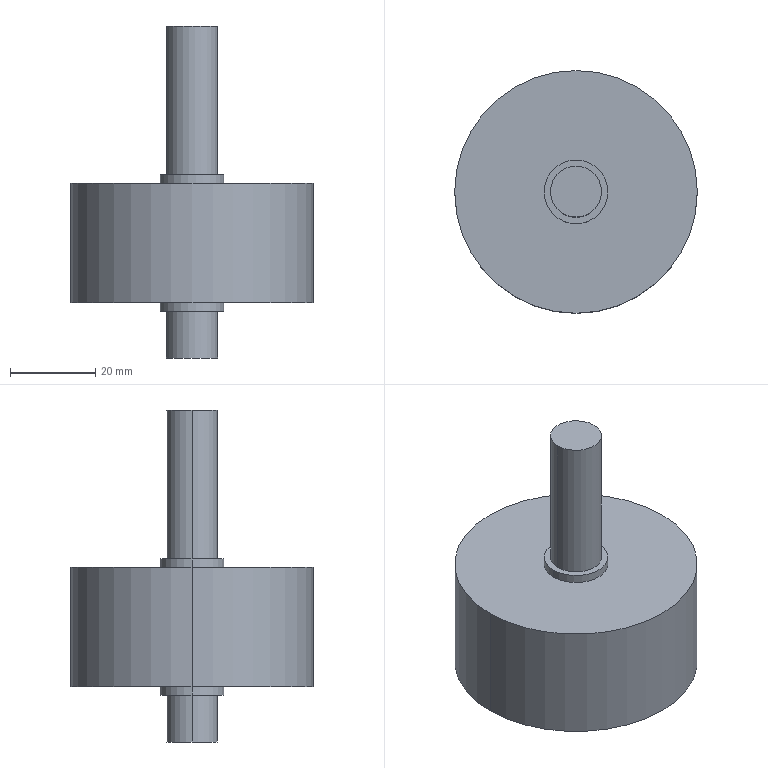Component | SolidWorks | --MA18S20041JR-SHuangGWDriveWheel-1 | 1 solid | 16 faces | box 57 x 57 x 78 mm | volume 77359 mm3 | cylinder 10 | plane 6 | commonest cylinder face diameters 12 x4 15 x4 57 x2
build123d program:
from build123d import *

# Parameters (mm, degrees)
SKETCH1_R           = 28.5
BOSS_EXTRUDE1_DEPTH = 28
SKETCH2_R           = 7.5
BOSS_EXTRUDE2_DEPTH = 2
BOSS_EXTRUDE3_START = 2
SKETCH3_R           = 7.5
BOSS_EXTRUDE3_DEPTH = 2
SKETCH4_R           = 6
BOSS_EXTRUDE4_DEPTH = 11
BOSS_EXTRUDE5_START = 35
SKETCH5_R           = 6
BOSS_EXTRUDE5_DEPTH = 35


with BuildPart() as part:
    # Sketch1 → Boss-Extrude1 (new body)
    with BuildSketch(Plane.XY):
        Circle(SKETCH1_R)
    extrude(amount=BOSS_EXTRUDE1_DEPTH)

    # Sketch2 → Boss-Extrude2 (add)
    with BuildSketch(Plane.XY.offset(28)):
        Circle(SKETCH2_R)
    extrude(amount=BOSS_EXTRUDE2_DEPTH)

    # Sketch3 → Boss-Extrude3 (add)
    with BuildSketch(Plane(origin=(0, 0, 0), x_dir=(-1, 0, 0), z_dir=(0, 0, -1)).offset(BOSS_EXTRUDE3_START)):
        with Locations(Location((0, 0, 0), (0, 0, 180))):
            Circle(SKETCH3_R)
    extrude(amount=-BOSS_EXTRUDE3_DEPTH)

    # Sketch4 → Boss-Extrude4 (add)
    with BuildSketch(Plane(origin=(0, 0, -2), x_dir=(-1, 0, 0), z_dir=(0, 0, -1))):
        Circle(SKETCH4_R)
    extrude(amount=BOSS_EXTRUDE4_DEPTH)

    # Sketch5 → Boss-Extrude5 (add)
    with BuildSketch(Plane.XY.offset(30).offset(BOSS_EXTRUDE5_START)):
        with Locations(Location((0, 0, 0), (0, 0, 180))):
            Circle(SKETCH5_R)
    extrude(amount=-BOSS_EXTRUDE5_DEPTH)


solid = part.part

# Placed as in the assembly
solid = solid.moved(Location((72.885, -33.301, 20), (0, 0, 0)))
STEP:
#1=COLOUR_RGB('',0.7922,0.8196,0.9333);
#2=FILL_AREA_STYLE_COLOUR('',#1);
#3=FILL_AREA_STYLE('',(#2));
#4=SURFACE_STYLE_FILL_AREA(#3);
#5=SURFACE_SIDE_STYLE('',(#4));
#6=SURFACE_STYLE_USAGE(.BOTH.,#5);
#7=PRESENTATION_STYLE_ASSIGNMENT((#6));
#8=CARTESIAN_POINT('',(3.106,-1.311,3.346));
#9=VERTEX_POINT('',#8);
#10=CARTESIAN_POINT('',(2.633,-1.311,3.346));
#11=VERTEX_POINT('',#10);
#12=CARTESIAN_POINT('',(2.869,-1.311,3.346));
#13=DIRECTION('',(0.,0.,1.));
#14=DIRECTION('',(1.,0.,0.));
#15=AXIS2_PLACEMENT_3D('',#12,#13,#14);
#16=CIRCLE('',#15,0.2362);
#17=EDGE_CURVE('',#9,#11,#16,.T.);
#18=ORIENTED_EDGE('',*,*,#17,.F.);
#19=CARTESIAN_POINT('',(3.106,-1.311,1.969));
#20=VERTEX_POINT('',#19);
#21=CARTESIAN_POINT('',(3.106,-1.311,3.346));
#22=DIRECTION('',(0.,0.,-1.));
#23=VECTOR('',#22,39.37);
#24=LINE('',#21,#23);
#25=EDGE_CURVE('',#9,#20,#24,.T.);
#26=ORIENTED_EDGE('',*,*,#25,.T.);
#27=CARTESIAN_POINT('',(2.633,-1.311,1.969));
#28=VERTEX_POINT('',#27);
#29=CARTESIAN_POINT('',(2.869,-1.311,1.969));
#30=DIRECTION('',(0.,0.,1.));
#31=DIRECTION('',(1.,0.,0.));
#32=AXIS2_PLACEMENT_3D('',#29,#30,#31);
#33=CIRCLE('',#32,0.2362);
#34=EDGE_CURVE('',#20,#28,#33,.T.);
#35=ORIENTED_EDGE('',*,*,#34,.T.);
#36=CARTESIAN_POINT('',(2.633,-1.311,3.346));
#37=DIRECTION('',(0.,0.,-1.));
#38=VECTOR('',#37,39.37);
#39=LINE('',#36,#38);
#40=EDGE_CURVE('',#11,#28,#39,.T.);
#41=ORIENTED_EDGE('',*,*,#40,.F.);
#42=EDGE_LOOP('',(#18,#26,#35,#41));
#43=FACE_OUTER_BOUND('',#42,.T.);
#44=CARTESIAN_POINT('',(2.869,-1.311,3.346));
#45=DIRECTION('',(0.,0.,-1.));
#46=DIRECTION('',(-1.,0.,0.));
#47=AXIS2_PLACEMENT_3D('',#44,#45,#46);
#48=CYLINDRICAL_SURFACE('',#47,0.2362);
#49=ADVANCED_FACE('',(#43),#48,.T.);
#50=CARTESIAN_POINT('',(2.633,-1.311,0.2756));
#51=VERTEX_POINT('',#50);
#52=CARTESIAN_POINT('',(3.106,-1.311,0.2756));
#53=VERTEX_POINT('',#52);
#54=CARTESIAN_POINT('',(2.869,-1.311,0.2756));
#55=DIRECTION('',(0.,0.,-1.));
#56=DIRECTION('',(-1.,0.,0.));
#57=AXIS2_PLACEMENT_3D('',#54,#55,#56);
#58=CIRCLE('',#57,0.2362);
#59=EDGE_CURVE('',#51,#53,#58,.T.);
#60=ORIENTED_EDGE('',*,*,#59,.F.);
#61=CARTESIAN_POINT('',(2.633,-1.311,0.7087));
#62=VERTEX_POINT('',#61);
#63=CARTESIAN_POINT('',(2.633,-1.311,0.2756));
#64=DIRECTION('',(0.,0.,1.));
#65=VECTOR('',#64,39.37);
#66=LINE('',#63,#65);
#67=EDGE_CURVE('',#51,#62,#66,.T.);
#68=ORIENTED_EDGE('',*,*,#67,.T.);
#69=CARTESIAN_POINT('',(3.106,-1.311,0.7087));
#70=VERTEX_POINT('',#69);
#71=CARTESIAN_POINT('',(2.869,-1.311,0.7087));
#72=DIRECTION('',(0.,0.,-1.));
#73=DIRECTION('',(-1.,0.,0.));
#74=AXIS2_PLACEMENT_3D('',#71,#72,#73);
#75=CIRCLE('',#74,0.2362);
#76=EDGE_CURVE('',#62,#70,#75,.T.);
#77=ORIENTED_EDGE('',*,*,#76,.T.);
#78=CARTESIAN_POINT('',(3.106,-1.311,0.2756));
#79=DIRECTION('',(0.,0.,1.));
#80=VECTOR('',#79,39.37);
#81=LINE('',#78,#80);
#82=EDGE_CURVE('',#53,#70,#81,.T.);
#83=ORIENTED_EDGE('',*,*,#82,.F.);
#84=EDGE_LOOP('',(#60,#68,#77,#83));
#85=FACE_OUTER_BOUND('',#84,.T.);
#86=CARTESIAN_POINT('',(2.869,-1.311,0.2756));
#87=DIRECTION('',(0.,0.,1.));
#88=DIRECTION('',(1.,0.,0.));
#89=AXIS2_PLACEMENT_3D('',#86,#87,#88);
#90=CYLINDRICAL_SURFACE('',#89,0.2362);
#91=ADVANCED_FACE('',(#85),#90,.T.);
#92=CARTESIAN_POINT('',(2.574,-1.311,0.7087));
#93=VERTEX_POINT('',#92);
#94=CARTESIAN_POINT('',(3.165,-1.311,0.7087));
#95=VERTEX_POINT('',#94);
#96=CARTESIAN_POINT('',(2.869,-1.311,0.7087));
#97=DIRECTION('',(0.,0.,-1.));
#98=DIRECTION('',(-1.,0.,0.));
#99=AXIS2_PLACEMENT_3D('',#96,#97,#98);
#100=CIRCLE('',#99,0.2953);
#101=EDGE_CURVE('',#93,#95,#100,.T.);
#102=ORIENTED_EDGE('',*,*,#101,.F.);
#103=CARTESIAN_POINT('',(2.574,-1.311,0.7874));
#104=VERTEX_POINT('',#103);
#105=CARTESIAN_POINT('',(2.574,-1.311,0.7087));
#106=DIRECTION('',(0.,0.,1.));
#107=VECTOR('',#106,39.37);
#108=LINE('',#105,#107);
#109=EDGE_CURVE('',#93,#104,#108,.T.);
#110=ORIENTED_EDGE('',*,*,#109,.T.);
#111=CARTESIAN_POINT('',(3.165,-1.311,0.7874));
#112=VERTEX_POINT('',#111);
#113=CARTESIAN_POINT('',(2.869,-1.311,0.7874));
#114=DIRECTION('',(0.,0.,-1.));
#115=DIRECTION('',(1.,0.,0.));
#116=AXIS2_PLACEMENT_3D('',#113,#114,#115);
#117=CIRCLE('',#116,0.2953);
#118=EDGE_CURVE('',#104,#112,#117,.T.);
#119=ORIENTED_EDGE('',*,*,#118,.T.);
#120=CARTESIAN_POINT('',(3.165,-1.311,0.7087));
#121=DIRECTION('',(0.,0.,1.));
#122=VECTOR('',#121,39.37);
#123=LINE('',#120,#122);
#124=EDGE_CURVE('',#95,#112,#123,.T.);
#125=ORIENTED_EDGE('',*,*,#124,.F.);
#126=EDGE_LOOP('',(#102,#110,#119,#125));
#127=FACE_OUTER_BOUND('',#126,.T.);
#128=CARTESIAN_POINT('',(2.869,-1.311,0.7087));
#129=DIRECTION('',(0.,0.,1.));
#130=DIRECTION('',(1.,0.,0.));
#131=AXIS2_PLACEMENT_3D('',#128,#129,#130);
#132=CYLINDRICAL_SURFACE('',#131,0.2953);
#133=ADVANCED_FACE('',(#127),#132,.T.);
#134=CARTESIAN_POINT('',(3.165,-1.311,1.969));
#135=VERTEX_POINT('',#134);
#136=CARTESIAN_POINT('',(2.574,-1.311,1.969));
#137=VERTEX_POINT('',#136);
#138=CARTESIAN_POINT('',(2.869,-1.311,1.969));
#139=DIRECTION('',(0.,0.,1.));
#140=DIRECTION('',(1.,0.,0.));
#141=AXIS2_PLACEMENT_3D('',#138,#139,#140);
#142=CIRCLE('',#141,0.2953);
#143=EDGE_CURVE('',#135,#137,#142,.T.);
#144=ORIENTED_EDGE('',*,*,#143,.F.);
#145=CARTESIAN_POINT('',(3.165,-1.311,1.89));
#146=VERTEX_POINT('',#145);
#147=CARTESIAN_POINT('',(3.165,-1.311,1.969));
#148=DIRECTION('',(0.,0.,-1.));
#149=VECTOR('',#148,39.37);
#150=LINE('',#147,#149);
#151=EDGE_CURVE('',#135,#146,#150,.T.);
#152=ORIENTED_EDGE('',*,*,#151,.T.);
#153=CARTESIAN_POINT('',(2.574,-1.311,1.89));
#154=VERTEX_POINT('',#153);
#155=CARTESIAN_POINT('',(2.869,-1.311,1.89));
#156=DIRECTION('',(0.,0.,1.));
#157=DIRECTION('',(1.,0.,0.));
#158=AXIS2_PLACEMENT_3D('',#155,#156,#157);
#159=CIRCLE('',#158,0.2953);
#160=EDGE_CURVE('',#146,#154,#159,.T.);
#161=ORIENTED_EDGE('',*,*,#160,.T.);
#162=CARTESIAN_POINT('',(2.574,-1.311,1.969));
#163=DIRECTION('',(0.,0.,-1.));
#164=VECTOR('',#163,39.37);
#165=LINE('',#162,#164);
#166=EDGE_CURVE('',#137,#154,#165,.T.);
#167=ORIENTED_EDGE('',*,*,#166,.F.);
#168=EDGE_LOOP('',(#144,#152,#161,#167));
#169=FACE_OUTER_BOUND('',#168,.T.);
#170=CARTESIAN_POINT('',(2.869,-1.311,1.969));
#171=DIRECTION('',(0.,0.,-1.));
#172=DIRECTION('',(-1.,0.,0.));
#173=AXIS2_PLACEMENT_3D('',#170,#171,#172);
#174=CYLINDRICAL_SURFACE('',#173,0.2953);
#175=ADVANCED_FACE('',(#169),#174,.T.);
#176=CARTESIAN_POINT('',(3.992,-1.311,1.89));
#177=VERTEX_POINT('',#176);
#178=CARTESIAN_POINT('',(1.747,-1.311,1.89));
#179=VERTEX_POINT('',#178);
#180=CARTESIAN_POINT('',(2.869,-1.311,1.89));
#181=DIRECTION('',(0.,0.,1.));
#182=DIRECTION('',(1.,0.,0.));
#183=AXIS2_PLACEMENT_3D('',#180,#181,#182);
#184=CIRCLE('',#183,1.122);
#185=EDGE_CURVE('',#177,#179,#184,.T.);
#186=ORIENTED_EDGE('',*,*,#185,.F.);
#187=CARTESIAN_POINT('',(3.992,-1.311,0.7874));
#188=VERTEX_POINT('',#187);
#189=CARTESIAN_POINT('',(3.992,-1.311,1.89));
#190=DIRECTION('',(0.,0.,-1.));
#191=VECTOR('',#190,39.37);
#192=LINE('',#189,#191);
#193=EDGE_CURVE('',#177,#188,#192,.T.);
#194=ORIENTED_EDGE('',*,*,#193,.T.);
#195=CARTESIAN_POINT('',(1.747,-1.311,0.7874));
#196=VERTEX_POINT('',#195);
#197=CARTESIAN_POINT('',(2.869,-1.311,0.7874));
#198=DIRECTION('',(0.,0.,1.));
#199=DIRECTION('',(1.,0.,0.));
#200=AXIS2_PLACEMENT_3D('',#197,#198,#199);
#201=CIRCLE('',#200,1.122);
#202=EDGE_CURVE('',#188,#196,#201,.T.);
#203=ORIENTED_EDGE('',*,*,#202,.T.);
#204=CARTESIAN_POINT('',(1.747,-1.311,1.89));
#205=DIRECTION('',(0.,0.,-1.));
#206=VECTOR('',#205,39.37);
#207=LINE('',#204,#206);
#208=EDGE_CURVE('',#179,#196,#207,.T.);
#209=ORIENTED_EDGE('',*,*,#208,.F.);
#210=EDGE_LOOP('',(#186,#194,#203,#209));
#211=FACE_OUTER_BOUND('',#210,.T.);
#212=CARTESIAN_POINT('',(2.869,-1.311,1.89));
#213=DIRECTION('',(0.,0.,-1.));
#214=DIRECTION('',(-1.,0.,0.));
#215=AXIS2_PLACEMENT_3D('',#212,#213,#214);
#216=CYLINDRICAL_SURFACE('',#215,1.122);
#217=ADVANCED_FACE('',(#211),#216,.T.);
#218=CARTESIAN_POINT('',(2.869,-1.311,1.969));
#219=DIRECTION('',(0.,0.,1.));
#220=DIRECTION('',(1.,0.,0.));
#221=AXIS2_PLACEMENT_3D('',#218,#219,#220);
#222=CIRCLE('',#221,0.2953);
#223=EDGE_CURVE('',#137,#135,#222,.T.);
#224=ORIENTED_EDGE('',*,*,#223,.T.);
#225=ORIENTED_EDGE('',*,*,#143,.T.);
#226=EDGE_LOOP('',(#224,#225));
#227=FACE_OUTER_BOUND('',#226,.T.);
#228=CARTESIAN_POINT('',(2.869,-1.311,1.969));
#229=DIRECTION('',(0.,0.,1.));
#230=DIRECTION('',(1.,0.,0.));
#231=AXIS2_PLACEMENT_3D('',#228,#229,#230);
#232=CIRCLE('',#231,0.2362);
#233=EDGE_CURVE('',#28,#20,#232,.T.);
#234=ORIENTED_EDGE('',*,*,#233,.F.);
#235=ORIENTED_EDGE('',*,*,#34,.F.);
#236=EDGE_LOOP('',(#234,#235));
#237=FACE_BOUND('',#236,.T.);
#238=CARTESIAN_POINT('',(2.869,-1.311,1.969));
#239=DIRECTION('',(0.,0.,1.));
#240=DIRECTION('',(1.,0.,0.));
#241=AXIS2_PLACEMENT_3D('',#238,#239,#240);
#242=PLANE('',#241);
#243=ADVANCED_FACE('',(#227,#237),#242,.T.);
#244=CARTESIAN_POINT('',(2.869,-1.311,0.7087));
#245=DIRECTION('',(0.,0.,-1.));
#246=DIRECTION('',(-1.,0.,0.));
#247=AXIS2_PLACEMENT_3D('',#244,#245,#246);
#248=CIRCLE('',#247,0.2953);
#249=EDGE_CURVE('',#95,#93,#248,.T.);
#250=ORIENTED_EDGE('',*,*,#249,.T.);
#251=ORIENTED_EDGE('',*,*,#101,.T.);
#252=EDGE_LOOP('',(#250,#251));
#253=FACE_OUTER_BOUND('',#252,.T.);
#254=CARTESIAN_POINT('',(2.869,-1.311,0.7087));
#255=DIRECTION('',(0.,0.,-1.));
#256=DIRECTION('',(-1.,0.,0.));
#257=AXIS2_PLACEMENT_3D('',#254,#255,#256);
#258=CIRCLE('',#257,0.2362);
#259=EDGE_CURVE('',#70,#62,#258,.T.);
#260=ORIENTED_EDGE('',*,*,#259,.F.);
#261=ORIENTED_EDGE('',*,*,#76,.F.);
#262=EDGE_LOOP('',(#260,#261));
#263=FACE_BOUND('',#262,.T.);
#264=CARTESIAN_POINT('',(2.869,-1.311,0.7087));
#265=DIRECTION('',(0.,0.,-1.));
#266=DIRECTION('',(-1.,0.,0.));
#267=AXIS2_PLACEMENT_3D('',#264,#265,#266);
#268=PLANE('',#267);
#269=ADVANCED_FACE('',(#253,#263),#268,.T.);
#270=CARTESIAN_POINT('',(2.869,-1.311,0.7874));
#271=DIRECTION('',(0.,0.,1.));
#272=DIRECTION('',(1.,0.,0.));
#273=AXIS2_PLACEMENT_3D('',#270,#271,#272);
#274=CIRCLE('',#273,1.122);
#275=EDGE_CURVE('',#196,#188,#274,.T.);
#276=ORIENTED_EDGE('',*,*,#275,.F.);
#277=ORIENTED_EDGE('',*,*,#202,.F.);
#278=EDGE_LOOP('',(#276,#277));
#279=FACE_OUTER_BOUND('',#278,.T.);
#280=CARTESIAN_POINT('',(2.869,-1.311,0.7874));
#281=DIRECTION('',(0.,0.,-1.));
#282=DIRECTION('',(1.,0.,0.));
#283=AXIS2_PLACEMENT_3D('',#280,#281,#282);
#284=CIRCLE('',#283,0.2953);
#285=EDGE_CURVE('',#112,#104,#284,.T.);
#286=ORIENTED_EDGE('',*,*,#285,.F.);
#287=ORIENTED_EDGE('',*,*,#118,.F.);
#288=EDGE_LOOP('',(#286,#287));
#289=FACE_BOUND('',#288,.T.);
#290=CARTESIAN_POINT('',(2.869,-1.311,0.7874));
#291=DIRECTION('',(0.,0.,1.));
#292=DIRECTION('',(1.,0.,0.));
#293=AXIS2_PLACEMENT_3D('',#290,#291,#292);
#294=PLANE('',#293);
#295=ADVANCED_FACE('',(#279,#289),#294,.F.);
#296=CARTESIAN_POINT('',(2.869,-1.311,1.89));
#297=DIRECTION('',(0.,0.,1.));
#298=DIRECTION('',(1.,0.,0.));
#299=AXIS2_PLACEMENT_3D('',#296,#297,#298);
#300=CIRCLE('',#299,1.122);
#301=EDGE_CURVE('',#179,#177,#300,.T.);
#302=ORIENTED_EDGE('',*,*,#301,.T.);
#303=ORIENTED_EDGE('',*,*,#185,.T.);
#304=EDGE_LOOP('',(#302,#303));
#305=FACE_OUTER_BOUND('',#304,.T.);
#306=CARTESIAN_POINT('',(2.869,-1.311,1.89));
#307=DIRECTION('',(0.,0.,1.));
#308=DIRECTION('',(1.,0.,0.));
#309=AXIS2_PLACEMENT_3D('',#306,#307,#308);
#310=CIRCLE('',#309,0.2953);
#311=EDGE_CURVE('',#154,#146,#310,.T.);
#312=ORIENTED_EDGE('',*,*,#311,.F.);
#313=ORIENTED_EDGE('',*,*,#160,.F.);
#314=EDGE_LOOP('',(#312,#313));
#315=FACE_BOUND('',#314,.T.);
#316=CARTESIAN_POINT('',(2.869,-1.311,1.89));
#317=DIRECTION('',(0.,0.,1.));
#318=DIRECTION('',(1.,0.,0.));
#319=AXIS2_PLACEMENT_3D('',#316,#317,#318);
#320=PLANE('',#319);
#321=ADVANCED_FACE('',(#305,#315),#320,.T.);
#322=ORIENTED_EDGE('',*,*,#193,.F.);
#323=ORIENTED_EDGE('',*,*,#301,.F.);
#324=ORIENTED_EDGE('',*,*,#208,.T.);
#325=ORIENTED_EDGE('',*,*,#275,.T.);
#326=EDGE_LOOP('',(#322,#323,#324,#325));
#327=FACE_OUTER_BOUND('',#326,.T.);
#328=CARTESIAN_POINT('',(2.869,-1.311,1.89));
#329=DIRECTION('',(0.,0.,-1.));
#330=DIRECTION('',(-1.,0.,0.));
#331=AXIS2_PLACEMENT_3D('',#328,#329,#330);
#332=CYLINDRICAL_SURFACE('',#331,1.122);
#333=ADVANCED_FACE('',(#327),#332,.T.);
#334=ORIENTED_EDGE('',*,*,#151,.F.);
#335=ORIENTED_EDGE('',*,*,#223,.F.);
#336=ORIENTED_EDGE('',*,*,#166,.T.);
#337=ORIENTED_EDGE('',*,*,#311,.T.);
#338=EDGE_LOOP('',(#334,#335,#336,#337));
#339=FACE_OUTER_BOUND('',#338,.T.);
#340=CARTESIAN_POINT('',(2.869,-1.311,1.969));
#341=DIRECTION('',(0.,0.,-1.));
#342=DIRECTION('',(-1.,0.,0.));
#343=AXIS2_PLACEMENT_3D('',#340,#341,#342);
#344=CYLINDRICAL_SURFACE('',#343,0.2953);
#345=ADVANCED_FACE('',(#339),#344,.T.);
#346=ORIENTED_EDGE('',*,*,#109,.F.);
#347=ORIENTED_EDGE('',*,*,#249,.F.);
#348=ORIENTED_EDGE('',*,*,#124,.T.);
#349=ORIENTED_EDGE('',*,*,#285,.T.);
#350=EDGE_LOOP('',(#346,#347,#348,#349));
#351=FACE_OUTER_BOUND('',#350,.T.);
#352=CARTESIAN_POINT('',(2.869,-1.311,0.7087));
#353=DIRECTION('',(0.,0.,1.));
#354=DIRECTION('',(1.,0.,0.));
#355=AXIS2_PLACEMENT_3D('',#352,#353,#354);
#356=CYLINDRICAL_SURFACE('',#355,0.2953);
#357=ADVANCED_FACE('',(#351),#356,.T.);
#358=ORIENTED_EDGE('',*,*,#67,.F.);
#359=CARTESIAN_POINT('',(2.869,-1.311,0.2756));
#360=DIRECTION('',(0.,0.,-1.));
#361=DIRECTION('',(-1.,0.,0.));
#362=AXIS2_PLACEMENT_3D('',#359,#360,#361);
#363=CIRCLE('',#362,0.2362);
#364=EDGE_CURVE('',#53,#51,#363,.T.);
#365=ORIENTED_EDGE('',*,*,#364,.F.);
#366=ORIENTED_EDGE('',*,*,#82,.T.);
#367=ORIENTED_EDGE('',*,*,#259,.T.);
#368=EDGE_LOOP('',(#358,#365,#366,#367));
#369=FACE_OUTER_BOUND('',#368,.T.);
#370=CARTESIAN_POINT('',(2.869,-1.311,0.2756));
#371=DIRECTION('',(0.,0.,1.));
#372=DIRECTION('',(1.,0.,0.));
#373=AXIS2_PLACEMENT_3D('',#370,#371,#372);
#374=CYLINDRICAL_SURFACE('',#373,0.2362);
#375=ADVANCED_FACE('',(#369),#374,.T.);
#376=ORIENTED_EDGE('',*,*,#364,.T.);
#377=ORIENTED_EDGE('',*,*,#59,.T.);
#378=EDGE_LOOP('',(#376,#377));
#379=FACE_OUTER_BOUND('',#378,.T.);
#380=CARTESIAN_POINT('',(2.869,-1.311,0.2756));
#381=DIRECTION('',(0.,0.,-1.));
#382=DIRECTION('',(-1.,0.,0.));
#383=AXIS2_PLACEMENT_3D('',#380,#381,#382);
#384=PLANE('',#383);
#385=ADVANCED_FACE('',(#379),#384,.T.);
#386=ORIENTED_EDGE('',*,*,#25,.F.);
#387=CARTESIAN_POINT('',(2.869,-1.311,3.346));
#388=DIRECTION('',(0.,0.,1.));
#389=DIRECTION('',(1.,0.,0.));
#390=AXIS2_PLACEMENT_3D('',#387,#388,#389);
#391=CIRCLE('',#390,0.2362);
#392=EDGE_CURVE('',#11,#9,#391,.T.);
#393=ORIENTED_EDGE('',*,*,#392,.F.);
#394=ORIENTED_EDGE('',*,*,#40,.T.);
#395=ORIENTED_EDGE('',*,*,#233,.T.);
#396=EDGE_LOOP('',(#386,#393,#394,#395));
#397=FACE_OUTER_BOUND('',#396,.T.);
#398=CARTESIAN_POINT('',(2.869,-1.311,3.346));
#399=DIRECTION('',(0.,0.,-1.));
#400=DIRECTION('',(-1.,0.,0.));
#401=AXIS2_PLACEMENT_3D('',#398,#399,#400);
#402=CYLINDRICAL_SURFACE('',#401,0.2362);
#403=ADVANCED_FACE('',(#397),#402,.T.);
#404=ORIENTED_EDGE('',*,*,#392,.T.);
#405=ORIENTED_EDGE('',*,*,#17,.T.);
#406=EDGE_LOOP('',(#404,#405));
#407=FACE_OUTER_BOUND('',#406,.T.);
#408=CARTESIAN_POINT('',(2.869,-1.311,3.346));
#409=DIRECTION('',(0.,0.,1.));
#410=DIRECTION('',(1.,0.,0.));
#411=AXIS2_PLACEMENT_3D('',#408,#409,#410);
#412=PLANE('',#411);
#413=ADVANCED_FACE('',(#407),#412,.T.);
#414=CLOSED_SHELL('',(#49,#91,#133,#175,#217,#243,#269,#295,#321,#333,#345,#357,#375,#385,#403,#413));
#415=MANIFOLD_SOLID_BREP('',#414);
#416=STYLED_ITEM('',(#7),#415);
#417=PRESENTATION_LAYER_ASSIGNMENT('','',(#416));
#418=CARTESIAN_POINT('',(0.,0.,0.));
#419=DIRECTION('',(0.,0.,1.));
#420=DIRECTION('',(1.,0.,0.));
#421=AXIS2_PLACEMENT_3D('',#418,#419,#420);
#422=(LENGTH_UNIT()NAMED_UNIT(*)SI_UNIT($,.METRE.));
#423=LENGTH_MEASURE_WITH_UNIT(LENGTH_MEASURE(0.0254),#422);
#424=DIMENSIONAL_EXPONENTS(1.,0.,0.,0.,0.,0.,0.);
#425=(CONVERSION_BASED_UNIT('',#423)LENGTH_UNIT()NAMED_UNIT(#424));
#426=UNCERTAINTY_MEASURE_WITH_UNIT(LENGTH_MEASURE(0.00001),#425,'','');
#427=(NAMED_UNIT(*)PLANE_ANGLE_UNIT()SI_UNIT($,.RADIAN.));
#428=(NAMED_UNIT(*)SI_UNIT($,.STERADIAN.)SOLID_ANGLE_UNIT());
#429=(GEOMETRIC_REPRESENTATION_CONTEXT(3)GLOBAL_UNCERTAINTY_ASSIGNED_CONTEXT((#426))GLOBAL_UNIT_ASSIGNED_CONTEXT((#425,#427,#428))REPRESENTATION_CONTEXT('',''));
#430=ADVANCED_BREP_SHAPE_REPRESENTATION('',(#415,#421),#429);
#431=(LENGTH_UNIT()NAMED_UNIT(*)SI_UNIT($,.METRE.));
#432=LENGTH_MEASURE_WITH_UNIT(LENGTH_MEASURE(0.0254),#431);
#433=DIMENSIONAL_EXPONENTS(1.,0.,0.,0.,0.,0.,0.);
#434=(CONVERSION_BASED_UNIT('',#432)LENGTH_UNIT()NAMED_UNIT(#433));
#435=UNCERTAINTY_MEASURE_WITH_UNIT(LENGTH_MEASURE(0.00001),#434,'','');
#436=(NAMED_UNIT(*)PLANE_ANGLE_UNIT()SI_UNIT($,.RADIAN.));
#437=(NAMED_UNIT(*)SI_UNIT($,.STERADIAN.)SOLID_ANGLE_UNIT());
#438=(GEOMETRIC_REPRESENTATION_CONTEXT(3)GLOBAL_UNCERTAINTY_ASSIGNED_CONTEXT((#435))GLOBAL_UNIT_ASSIGNED_CONTEXT((#434,#436,#437))REPRESENTATION_CONTEXT('',''));
#439=MECHANICAL_DESIGN_GEOMETRIC_PRESENTATION_REPRESENTATION('',(#416),#438);